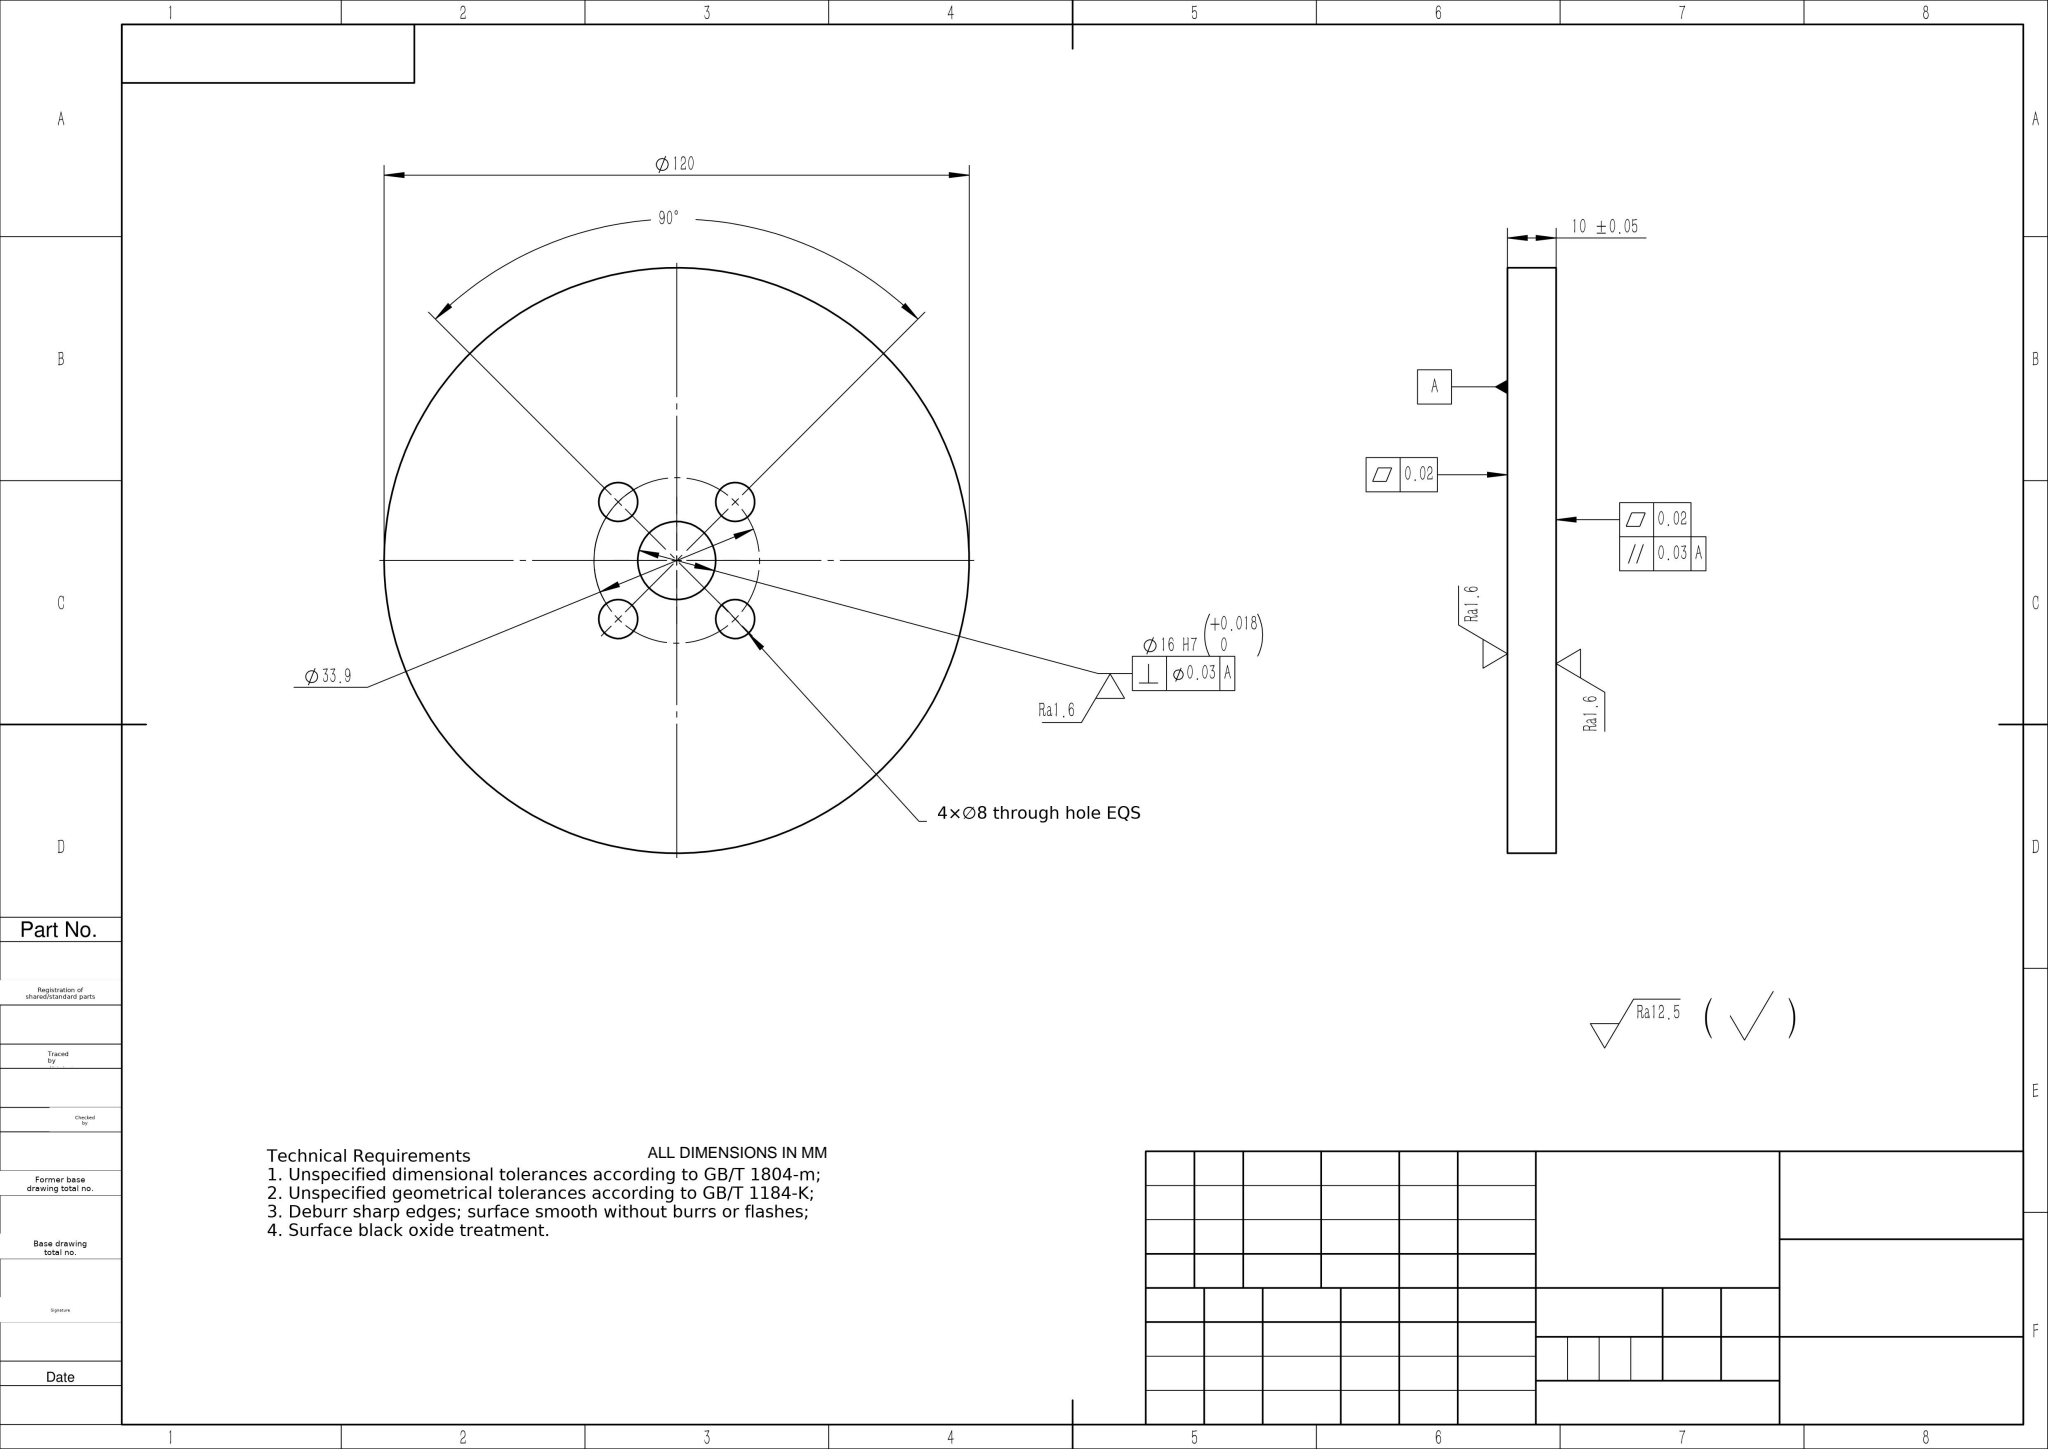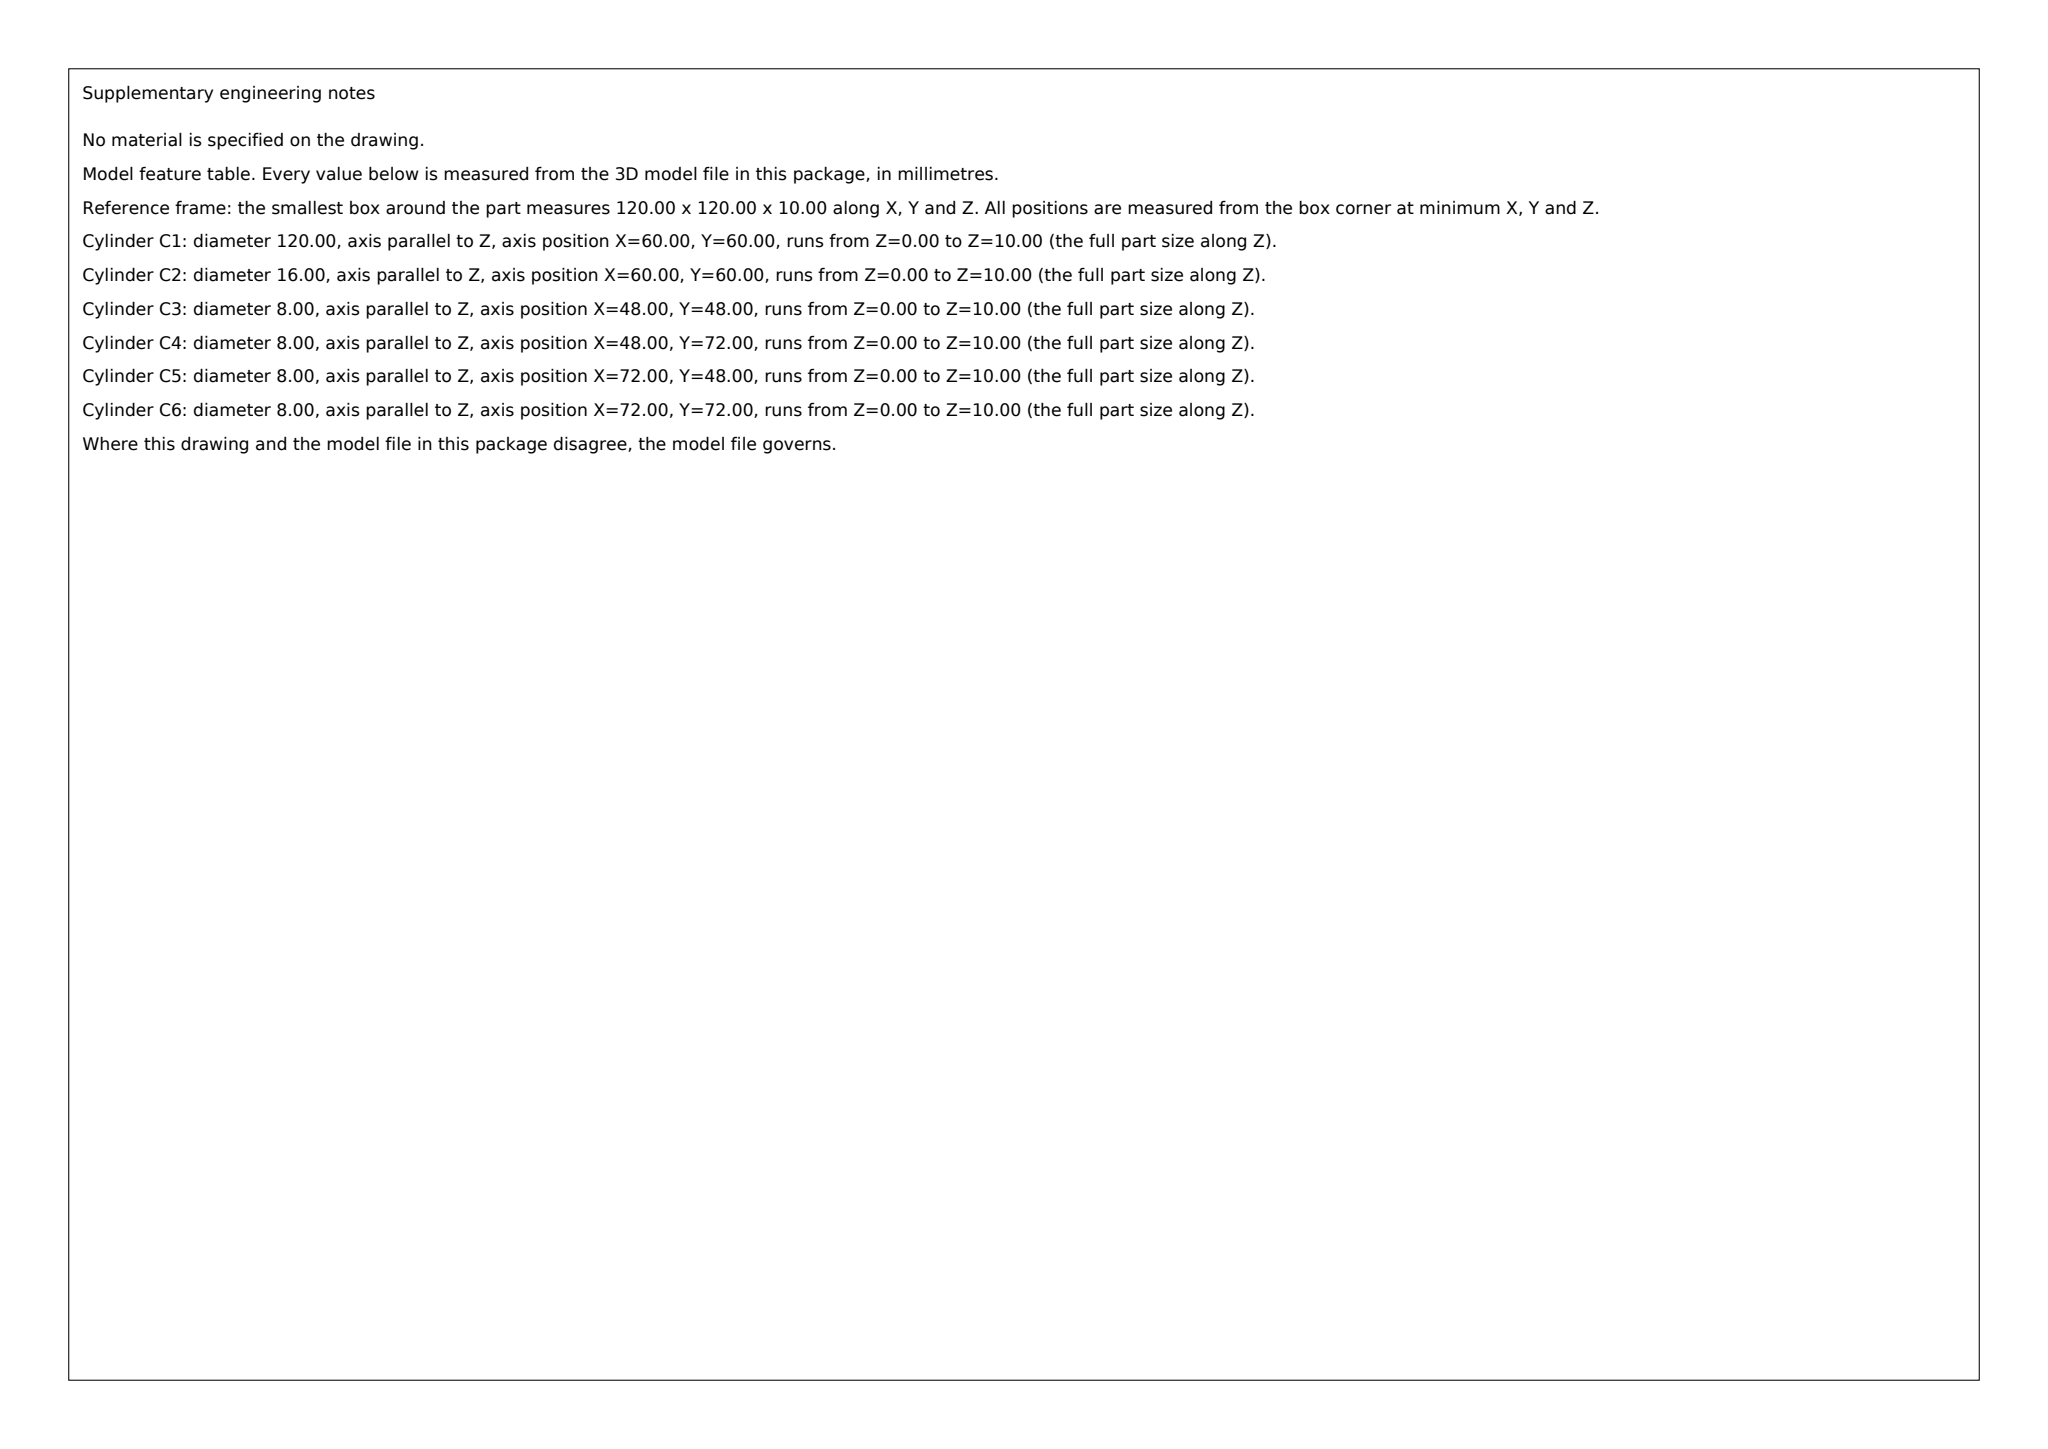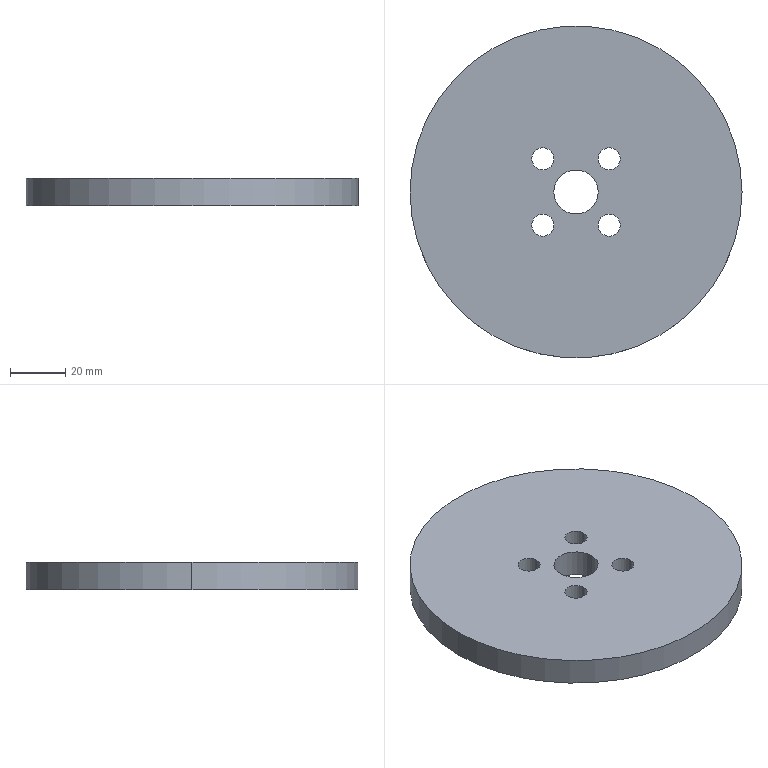Part | SolidWorks | mm | 1 solid | 14 faces | box 120 x 120 x 10 mm | volume 109076 mm3 | cylinder 12 | plane 2 | commonest cylinder face diameters 8 x8 16 x2 120 x2
build123d program:
from build123d import *

# Parameters (mm, degrees)
SKETCH1_R           = 20
BOSS_EXTRUDE1_DEPTH = 5
SKETCH2_R           = 30
BOSS_EXTRUDE2_DEPTH = 5
CUT_EXTRUDE1_REACH  = 44.72
SKETCH3_R           = 2
CUT_EXTRUDE3_REACH  = 44.72
SKETCH5_R           = 4
SCALE1_SCALE        = 2


with BuildPart() as part:
    # Sketch1 → Boss-Extrude1 (new body)
    with BuildSketch(Plane.XY):
        Circle(SKETCH1_R)
    extrude(amount=BOSS_EXTRUDE1_DEPTH)

    # Sketch2 → Boss-Extrude2 (add)
    with BuildSketch(Plane.XY.offset(5)):
        Circle(SKETCH2_R)
    extrude(amount=-BOSS_EXTRUDE2_DEPTH)

    # Sketch3 → Cut-Extrude1 (cut, up to next)
    with BuildSketch(Plane.XY.offset(5), mode=Mode.PRIVATE) as cut_extrude1_sk1:
        with Locations((-6, 6)):
            Circle(SKETCH3_R)
    cut_extrude1_tool1 = extrude(cut_extrude1_sk1.sketch, amount=-CUT_EXTRUDE1_REACH, mode=Mode.PRIVATE) & part.part
    # Sketch3 → Cut-Extrude1 (cut, up to next)
    with BuildSketch(Plane.XY.offset(5), mode=Mode.PRIVATE) as cut_extrude1_sk2:
        with Locations((-6, -6)):
            Circle(SKETCH3_R)
    cut_extrude1_tool2 = extrude(cut_extrude1_sk2.sketch, amount=-CUT_EXTRUDE1_REACH, mode=Mode.PRIVATE) & part.part
    # Sketch3 → Cut-Extrude1 (cut, up to next)
    with BuildSketch(Plane.XY.offset(5), mode=Mode.PRIVATE) as cut_extrude1_sk3:
        with Locations((6, -6)):
            Circle(SKETCH3_R)
    cut_extrude1_tool3 = extrude(cut_extrude1_sk3.sketch, amount=-CUT_EXTRUDE1_REACH, mode=Mode.PRIVATE) & part.part
    # Sketch3 → Cut-Extrude1 (cut, up to next)
    with BuildSketch(Plane.XY.offset(5), mode=Mode.PRIVATE) as cut_extrude1_sk4:
        with Locations((6, 6)):
            Circle(SKETCH3_R)
    cut_extrude1_tool4 = extrude(cut_extrude1_sk4.sketch, amount=-CUT_EXTRUDE1_REACH, mode=Mode.PRIVATE) & part.part
    add(cut_extrude1_tool1.solids().sort_by_distance((-6, 6, 5))[0], mode=Mode.SUBTRACT)
    add(cut_extrude1_tool2.solids().sort_by_distance((-6, -6, 5))[0], mode=Mode.SUBTRACT)
    add(cut_extrude1_tool3.solids().sort_by_distance((6, -6, 5))[0], mode=Mode.SUBTRACT)
    add(cut_extrude1_tool4.solids().sort_by_distance((6, 6, 5))[0], mode=Mode.SUBTRACT)

    # Sketch5 → Cut-Extrude3 (cut, up to next)
    with BuildSketch(Plane(origin=(0, 0, 0), x_dir=(-1, 0, 0), z_dir=(0, 0, -1)), mode=Mode.PRIVATE) as cut_extrude3_sk1:
        Circle(SKETCH5_R)
    cut_extrude3_tool1 = extrude(cut_extrude3_sk1.sketch, amount=-CUT_EXTRUDE3_REACH, mode=Mode.PRIVATE) & part.part
    add(cut_extrude3_tool1.solids().sort_by_distance((0, 0, 0))[0], mode=Mode.SUBTRACT)


with BuildPart() as part_1:
    # Scale1: scaled about (0, 0, 2.5)
    add(part.part.scale(SCALE1_SCALE).moved(Location((0, 0, -2.5))))


solid = part_1.part
STEP:
#1=CARTESIAN_POINT('',(8.,0.,7.5));
#2=VERTEX_POINT('',#1);
#3=CARTESIAN_POINT('',(-8.,0.,7.5));
#4=VERTEX_POINT('',#3);
#5=CARTESIAN_POINT('',(0.,0.,7.5));
#6=DIRECTION('',(0.,-0.,-1.));
#7=DIRECTION('',(1.,-0.,0.));
#8=AXIS2_PLACEMENT_3D('',#5,#6,#7);
#9=CIRCLE('',#8,8.);
#10=EDGE_CURVE('',#2,#4,#9,.T.);
#11=ORIENTED_EDGE('',*,*,#10,.F.);
#12=CARTESIAN_POINT('',(8.,0.,-2.5));
#13=VERTEX_POINT('',#12);
#14=CARTESIAN_POINT('',(8.,0.,7.502));
#15=DIRECTION('',(0.,-0.,-1.));
#16=VECTOR('',#15,1000.);
#17=LINE('',#14,#16);
#18=EDGE_CURVE('',#2,#13,#17,.T.);
#19=ORIENTED_EDGE('',*,*,#18,.T.);
#20=CARTESIAN_POINT('',(-8.,0.,-2.5));
#21=VERTEX_POINT('',#20);
#22=CARTESIAN_POINT('',(0.,0.,-2.5));
#23=DIRECTION('',(0.,-0.,-1.));
#24=DIRECTION('',(-1.,0.,0.));
#25=AXIS2_PLACEMENT_3D('',#22,#23,#24);
#26=CIRCLE('',#25,8.);
#27=EDGE_CURVE('',#13,#21,#26,.T.);
#28=ORIENTED_EDGE('',*,*,#27,.T.);
#29=CARTESIAN_POINT('',(-8.,0.,7.502));
#30=DIRECTION('',(0.,-0.,-1.));
#31=VECTOR('',#30,1000.);
#32=LINE('',#29,#31);
#33=EDGE_CURVE('',#4,#21,#32,.T.);
#34=ORIENTED_EDGE('',*,*,#33,.F.);
#35=EDGE_LOOP('',(#11,#19,#28,#34));
#36=FACE_OUTER_BOUND('',#35,.T.);
#37=CARTESIAN_POINT('',(0.,0.,7.502));
#38=DIRECTION('',(0.,-0.,-1.));
#39=DIRECTION('',(-1.,0.,0.));
#40=AXIS2_PLACEMENT_3D('',#37,#38,#39);
#41=CYLINDRICAL_SURFACE('',#40,8.);
#42=ADVANCED_FACE('',(#36),#41,.F.);
#43=CARTESIAN_POINT('',(16.,12.,-2.5));
#44=VERTEX_POINT('',#43);
#45=CARTESIAN_POINT('',(8.,12.,-2.5));
#46=VERTEX_POINT('',#45);
#47=CARTESIAN_POINT('',(12.,12.,-2.5));
#48=DIRECTION('',(0.,-0.,-1.));
#49=DIRECTION('',(1.,0.,0.));
#50=AXIS2_PLACEMENT_3D('',#47,#48,#49);
#51=CIRCLE('',#50,4.);
#52=EDGE_CURVE('',#44,#46,#51,.T.);
#53=ORIENTED_EDGE('',*,*,#52,.T.);
#54=CARTESIAN_POINT('',(8.,12.,7.5));
#55=VERTEX_POINT('',#54);
#56=CARTESIAN_POINT('',(8.,12.,-2.502));
#57=DIRECTION('',(-0.,0.,1.));
#58=VECTOR('',#57,1000.);
#59=LINE('',#56,#58);
#60=EDGE_CURVE('',#46,#55,#59,.T.);
#61=ORIENTED_EDGE('',*,*,#60,.T.);
#62=CARTESIAN_POINT('',(16.,12.,7.5));
#63=VERTEX_POINT('',#62);
#64=CARTESIAN_POINT('',(12.,12.,7.5));
#65=DIRECTION('',(-0.,0.,1.));
#66=DIRECTION('',(1.,0.,0.));
#67=AXIS2_PLACEMENT_3D('',#64,#65,#66);
#68=CIRCLE('',#67,4.);
#69=EDGE_CURVE('',#55,#63,#68,.T.);
#70=ORIENTED_EDGE('',*,*,#69,.T.);
#71=CARTESIAN_POINT('',(16.,12.,-2.502));
#72=DIRECTION('',(-0.,0.,1.));
#73=VECTOR('',#72,1000.);
#74=LINE('',#71,#73);
#75=EDGE_CURVE('',#44,#63,#74,.T.);
#76=ORIENTED_EDGE('',*,*,#75,.F.);
#77=EDGE_LOOP('',(#53,#61,#70,#76));
#78=FACE_OUTER_BOUND('',#77,.T.);
#79=CARTESIAN_POINT('',(12.,12.,-2.502));
#80=DIRECTION('',(-0.,0.,1.));
#81=DIRECTION('',(1.,0.,0.));
#82=AXIS2_PLACEMENT_3D('',#79,#80,#81);
#83=CYLINDRICAL_SURFACE('',#82,4.);
#84=ADVANCED_FACE('',(#78),#83,.F.);
#85=CARTESIAN_POINT('',(16.,-12.,-2.5));
#86=VERTEX_POINT('',#85);
#87=CARTESIAN_POINT('',(8.,-12.,-2.5));
#88=VERTEX_POINT('',#87);
#89=CARTESIAN_POINT('',(12.,-12.,-2.5));
#90=DIRECTION('',(0.,-0.,-1.));
#91=DIRECTION('',(1.,0.,0.));
#92=AXIS2_PLACEMENT_3D('',#89,#90,#91);
#93=CIRCLE('',#92,4.);
#94=EDGE_CURVE('',#86,#88,#93,.T.);
#95=ORIENTED_EDGE('',*,*,#94,.T.);
#96=CARTESIAN_POINT('',(8.,-12.,7.5));
#97=VERTEX_POINT('',#96);
#98=CARTESIAN_POINT('',(8.,-12.,-2.502));
#99=DIRECTION('',(-0.,0.,1.));
#100=VECTOR('',#99,1000.);
#101=LINE('',#98,#100);
#102=EDGE_CURVE('',#88,#97,#101,.T.);
#103=ORIENTED_EDGE('',*,*,#102,.T.);
#104=CARTESIAN_POINT('',(16.,-12.,7.5));
#105=VERTEX_POINT('',#104);
#106=CARTESIAN_POINT('',(12.,-12.,7.5));
#107=DIRECTION('',(-0.,0.,1.));
#108=DIRECTION('',(1.,0.,0.));
#109=AXIS2_PLACEMENT_3D('',#106,#107,#108);
#110=CIRCLE('',#109,4.);
#111=EDGE_CURVE('',#97,#105,#110,.T.);
#112=ORIENTED_EDGE('',*,*,#111,.T.);
#113=CARTESIAN_POINT('',(16.,-12.,-2.502));
#114=DIRECTION('',(-0.,0.,1.));
#115=VECTOR('',#114,1000.);
#116=LINE('',#113,#115);
#117=EDGE_CURVE('',#86,#105,#116,.T.);
#118=ORIENTED_EDGE('',*,*,#117,.F.);
#119=EDGE_LOOP('',(#95,#103,#112,#118));
#120=FACE_OUTER_BOUND('',#119,.T.);
#121=CARTESIAN_POINT('',(12.,-12.,-2.502));
#122=DIRECTION('',(-0.,0.,1.));
#123=DIRECTION('',(1.,0.,0.));
#124=AXIS2_PLACEMENT_3D('',#121,#122,#123);
#125=CYLINDRICAL_SURFACE('',#124,4.);
#126=ADVANCED_FACE('',(#120),#125,.F.);
#127=CARTESIAN_POINT('',(-8.,-12.,-2.5));
#128=VERTEX_POINT('',#127);
#129=CARTESIAN_POINT('',(-16.,-12.,-2.5));
#130=VERTEX_POINT('',#129);
#131=CARTESIAN_POINT('',(-12.,-12.,-2.5));
#132=DIRECTION('',(0.,-0.,-1.));
#133=DIRECTION('',(1.,0.,0.));
#134=AXIS2_PLACEMENT_3D('',#131,#132,#133);
#135=CIRCLE('',#134,4.);
#136=EDGE_CURVE('',#128,#130,#135,.T.);
#137=ORIENTED_EDGE('',*,*,#136,.T.);
#138=CARTESIAN_POINT('',(-16.,-12.,7.5));
#139=VERTEX_POINT('',#138);
#140=CARTESIAN_POINT('',(-16.,-12.,-2.502));
#141=DIRECTION('',(-0.,0.,1.));
#142=VECTOR('',#141,1000.);
#143=LINE('',#140,#142);
#144=EDGE_CURVE('',#130,#139,#143,.T.);
#145=ORIENTED_EDGE('',*,*,#144,.T.);
#146=CARTESIAN_POINT('',(-8.,-12.,7.5));
#147=VERTEX_POINT('',#146);
#148=CARTESIAN_POINT('',(-12.,-12.,7.5));
#149=DIRECTION('',(-0.,0.,1.));
#150=DIRECTION('',(1.,0.,0.));
#151=AXIS2_PLACEMENT_3D('',#148,#149,#150);
#152=CIRCLE('',#151,4.);
#153=EDGE_CURVE('',#139,#147,#152,.T.);
#154=ORIENTED_EDGE('',*,*,#153,.T.);
#155=CARTESIAN_POINT('',(-8.,-12.,-2.502));
#156=DIRECTION('',(-0.,0.,1.));
#157=VECTOR('',#156,1000.);
#158=LINE('',#155,#157);
#159=EDGE_CURVE('',#128,#147,#158,.T.);
#160=ORIENTED_EDGE('',*,*,#159,.F.);
#161=EDGE_LOOP('',(#137,#145,#154,#160));
#162=FACE_OUTER_BOUND('',#161,.T.);
#163=CARTESIAN_POINT('',(-12.,-12.,-2.502));
#164=DIRECTION('',(-0.,0.,1.));
#165=DIRECTION('',(1.,0.,0.));
#166=AXIS2_PLACEMENT_3D('',#163,#164,#165);
#167=CYLINDRICAL_SURFACE('',#166,4.);
#168=ADVANCED_FACE('',(#162),#167,.F.);
#169=CARTESIAN_POINT('',(-8.,12.,-2.5));
#170=VERTEX_POINT('',#169);
#171=CARTESIAN_POINT('',(-16.,12.,-2.5));
#172=VERTEX_POINT('',#171);
#173=CARTESIAN_POINT('',(-12.,12.,-2.5));
#174=DIRECTION('',(0.,-0.,-1.));
#175=DIRECTION('',(1.,0.,0.));
#176=AXIS2_PLACEMENT_3D('',#173,#174,#175);
#177=CIRCLE('',#176,4.);
#178=EDGE_CURVE('',#170,#172,#177,.T.);
#179=ORIENTED_EDGE('',*,*,#178,.T.);
#180=CARTESIAN_POINT('',(-16.,12.,7.5));
#181=VERTEX_POINT('',#180);
#182=CARTESIAN_POINT('',(-16.,12.,-2.502));
#183=DIRECTION('',(-0.,0.,1.));
#184=VECTOR('',#183,1000.);
#185=LINE('',#182,#184);
#186=EDGE_CURVE('',#172,#181,#185,.T.);
#187=ORIENTED_EDGE('',*,*,#186,.T.);
#188=CARTESIAN_POINT('',(-8.,12.,7.5));
#189=VERTEX_POINT('',#188);
#190=CARTESIAN_POINT('',(-12.,12.,7.5));
#191=DIRECTION('',(-0.,0.,1.));
#192=DIRECTION('',(1.,0.,0.));
#193=AXIS2_PLACEMENT_3D('',#190,#191,#192);
#194=CIRCLE('',#193,4.);
#195=EDGE_CURVE('',#181,#189,#194,.T.);
#196=ORIENTED_EDGE('',*,*,#195,.T.);
#197=CARTESIAN_POINT('',(-8.,12.,-2.502));
#198=DIRECTION('',(-0.,0.,1.));
#199=VECTOR('',#198,1000.);
#200=LINE('',#197,#199);
#201=EDGE_CURVE('',#170,#189,#200,.T.);
#202=ORIENTED_EDGE('',*,*,#201,.F.);
#203=EDGE_LOOP('',(#179,#187,#196,#202));
#204=FACE_OUTER_BOUND('',#203,.T.);
#205=CARTESIAN_POINT('',(-12.,12.,-2.502));
#206=DIRECTION('',(-0.,0.,1.));
#207=DIRECTION('',(1.,0.,0.));
#208=AXIS2_PLACEMENT_3D('',#205,#206,#207);
#209=CYLINDRICAL_SURFACE('',#208,4.);
#210=ADVANCED_FACE('',(#204),#209,.F.);
#211=CARTESIAN_POINT('',(60.,-0.,-2.5));
#212=VERTEX_POINT('',#211);
#213=CARTESIAN_POINT('',(-60.,0.,-2.5));
#214=VERTEX_POINT('',#213);
#215=CARTESIAN_POINT('',(0.,0.,-2.5));
#216=DIRECTION('',(-0.,0.,1.));
#217=DIRECTION('',(1.,-0.,0.));
#218=AXIS2_PLACEMENT_3D('',#215,#216,#217);
#219=CIRCLE('',#218,60.);
#220=EDGE_CURVE('',#212,#214,#219,.T.);
#221=ORIENTED_EDGE('',*,*,#220,.T.);
#222=CARTESIAN_POINT('',(-60.,0.,7.5));
#223=VERTEX_POINT('',#222);
#224=CARTESIAN_POINT('',(-60.,0.,-2.5));
#225=DIRECTION('',(-0.,0.,1.));
#226=VECTOR('',#225,1000.);
#227=LINE('',#224,#226);
#228=EDGE_CURVE('',#214,#223,#227,.T.);
#229=ORIENTED_EDGE('',*,*,#228,.T.);
#230=CARTESIAN_POINT('',(60.,-0.,7.5));
#231=VERTEX_POINT('',#230);
#232=CARTESIAN_POINT('',(0.,0.,7.5));
#233=DIRECTION('',(-0.,0.,1.));
#234=DIRECTION('',(1.,-0.,0.));
#235=AXIS2_PLACEMENT_3D('',#232,#233,#234);
#236=CIRCLE('',#235,60.);
#237=EDGE_CURVE('',#231,#223,#236,.T.);
#238=ORIENTED_EDGE('',*,*,#237,.F.);
#239=CARTESIAN_POINT('',(60.,-0.,-2.5));
#240=DIRECTION('',(-0.,0.,1.));
#241=VECTOR('',#240,1000.);
#242=LINE('',#239,#241);
#243=EDGE_CURVE('',#212,#231,#242,.T.);
#244=ORIENTED_EDGE('',*,*,#243,.F.);
#245=EDGE_LOOP('',(#221,#229,#238,#244));
#246=FACE_OUTER_BOUND('',#245,.T.);
#247=CARTESIAN_POINT('',(0.,0.,-2.5));
#248=DIRECTION('',(-0.,0.,1.));
#249=DIRECTION('',(1.,-0.,0.));
#250=AXIS2_PLACEMENT_3D('',#247,#248,#249);
#251=CYLINDRICAL_SURFACE('',#250,60.);
#252=ADVANCED_FACE('',(#246),#251,.T.);
#253=CARTESIAN_POINT('',(0.,0.,-2.5));
#254=DIRECTION('',(0.,-0.,-1.));
#255=DIRECTION('',(-1.,0.,0.));
#256=AXIS2_PLACEMENT_3D('',#253,#254,#255);
#257=CIRCLE('',#256,8.);
#258=EDGE_CURVE('',#21,#13,#257,.T.);
#259=ORIENTED_EDGE('',*,*,#258,.F.);
#260=ORIENTED_EDGE('',*,*,#27,.F.);
#261=EDGE_LOOP('',(#259,#260));
#262=FACE_BOUND('',#261,.T.);
#263=ORIENTED_EDGE('',*,*,#52,.F.);
#264=CARTESIAN_POINT('',(12.,12.,-2.5));
#265=DIRECTION('',(0.,-0.,-1.));
#266=DIRECTION('',(1.,0.,0.));
#267=AXIS2_PLACEMENT_3D('',#264,#265,#266);
#268=CIRCLE('',#267,4.);
#269=EDGE_CURVE('',#46,#44,#268,.T.);
#270=ORIENTED_EDGE('',*,*,#269,.F.);
#271=EDGE_LOOP('',(#263,#270));
#272=FACE_BOUND('',#271,.T.);
#273=ORIENTED_EDGE('',*,*,#94,.F.);
#274=CARTESIAN_POINT('',(12.,-12.,-2.5));
#275=DIRECTION('',(0.,-0.,-1.));
#276=DIRECTION('',(1.,0.,0.));
#277=AXIS2_PLACEMENT_3D('',#274,#275,#276);
#278=CIRCLE('',#277,4.);
#279=EDGE_CURVE('',#88,#86,#278,.T.);
#280=ORIENTED_EDGE('',*,*,#279,.F.);
#281=EDGE_LOOP('',(#273,#280));
#282=FACE_BOUND('',#281,.T.);
#283=ORIENTED_EDGE('',*,*,#136,.F.);
#284=CARTESIAN_POINT('',(-12.,-12.,-2.5));
#285=DIRECTION('',(0.,-0.,-1.));
#286=DIRECTION('',(1.,0.,0.));
#287=AXIS2_PLACEMENT_3D('',#284,#285,#286);
#288=CIRCLE('',#287,4.);
#289=EDGE_CURVE('',#130,#128,#288,.T.);
#290=ORIENTED_EDGE('',*,*,#289,.F.);
#291=EDGE_LOOP('',(#283,#290));
#292=FACE_BOUND('',#291,.T.);
#293=ORIENTED_EDGE('',*,*,#178,.F.);
#294=CARTESIAN_POINT('',(-12.,12.,-2.5));
#295=DIRECTION('',(0.,-0.,-1.));
#296=DIRECTION('',(1.,0.,0.));
#297=AXIS2_PLACEMENT_3D('',#294,#295,#296);
#298=CIRCLE('',#297,4.);
#299=EDGE_CURVE('',#172,#170,#298,.T.);
#300=ORIENTED_EDGE('',*,*,#299,.F.);
#301=EDGE_LOOP('',(#293,#300));
#302=FACE_BOUND('',#301,.T.);
#303=ORIENTED_EDGE('',*,*,#220,.F.);
#304=CARTESIAN_POINT('',(0.,0.,-2.5));
#305=DIRECTION('',(-0.,0.,1.));
#306=DIRECTION('',(1.,-0.,0.));
#307=AXIS2_PLACEMENT_3D('',#304,#305,#306);
#308=CIRCLE('',#307,60.);
#309=EDGE_CURVE('',#214,#212,#308,.T.);
#310=ORIENTED_EDGE('',*,*,#309,.F.);
#311=EDGE_LOOP('',(#303,#310));
#312=FACE_OUTER_BOUND('',#311,.T.);
#313=CARTESIAN_POINT('',(0.,0.,-2.5));
#314=DIRECTION('',(0.,0.,1.));
#315=DIRECTION('',(1.,-0.,-0.));
#316=AXIS2_PLACEMENT_3D('',#313,#314,#315);
#317=PLANE('',#316);
#318=ADVANCED_FACE('',(#262,#272,#282,#292,#302,#312),#317,.F.);
#319=ORIENTED_EDGE('',*,*,#228,.F.);
#320=ORIENTED_EDGE('',*,*,#309,.T.);
#321=ORIENTED_EDGE('',*,*,#243,.T.);
#322=CARTESIAN_POINT('',(0.,0.,7.5));
#323=DIRECTION('',(-0.,0.,1.));
#324=DIRECTION('',(1.,-0.,0.));
#325=AXIS2_PLACEMENT_3D('',#322,#323,#324);
#326=CIRCLE('',#325,60.);
#327=EDGE_CURVE('',#223,#231,#326,.T.);
#328=ORIENTED_EDGE('',*,*,#327,.F.);
#329=EDGE_LOOP('',(#319,#320,#321,#328));
#330=FACE_OUTER_BOUND('',#329,.T.);
#331=CARTESIAN_POINT('',(0.,0.,-2.5));
#332=DIRECTION('',(-0.,0.,1.));
#333=DIRECTION('',(1.,-0.,0.));
#334=AXIS2_PLACEMENT_3D('',#331,#332,#333);
#335=CYLINDRICAL_SURFACE('',#334,60.);
#336=ADVANCED_FACE('',(#330),#335,.T.);
#337=CARTESIAN_POINT('',(0.,0.,7.5));
#338=DIRECTION('',(0.,-0.,-1.));
#339=DIRECTION('',(1.,-0.,0.));
#340=AXIS2_PLACEMENT_3D('',#337,#338,#339);
#341=CIRCLE('',#340,8.);
#342=EDGE_CURVE('',#4,#2,#341,.T.);
#343=ORIENTED_EDGE('',*,*,#342,.T.);
#344=ORIENTED_EDGE('',*,*,#10,.T.);
#345=EDGE_LOOP('',(#343,#344));
#346=FACE_BOUND('',#345,.T.);
#347=CARTESIAN_POINT('',(12.,12.,7.5));
#348=DIRECTION('',(-0.,0.,1.));
#349=DIRECTION('',(1.,0.,0.));
#350=AXIS2_PLACEMENT_3D('',#347,#348,#349);
#351=CIRCLE('',#350,4.);
#352=EDGE_CURVE('',#63,#55,#351,.T.);
#353=ORIENTED_EDGE('',*,*,#352,.F.);
#354=ORIENTED_EDGE('',*,*,#69,.F.);
#355=EDGE_LOOP('',(#353,#354));
#356=FACE_BOUND('',#355,.T.);
#357=CARTESIAN_POINT('',(12.,-12.,7.5));
#358=DIRECTION('',(-0.,0.,1.));
#359=DIRECTION('',(1.,0.,0.));
#360=AXIS2_PLACEMENT_3D('',#357,#358,#359);
#361=CIRCLE('',#360,4.);
#362=EDGE_CURVE('',#105,#97,#361,.T.);
#363=ORIENTED_EDGE('',*,*,#362,.F.);
#364=ORIENTED_EDGE('',*,*,#111,.F.);
#365=EDGE_LOOP('',(#363,#364));
#366=FACE_BOUND('',#365,.T.);
#367=CARTESIAN_POINT('',(-12.,-12.,7.5));
#368=DIRECTION('',(-0.,0.,1.));
#369=DIRECTION('',(1.,0.,0.));
#370=AXIS2_PLACEMENT_3D('',#367,#368,#369);
#371=CIRCLE('',#370,4.);
#372=EDGE_CURVE('',#147,#139,#371,.T.);
#373=ORIENTED_EDGE('',*,*,#372,.F.);
#374=ORIENTED_EDGE('',*,*,#153,.F.);
#375=EDGE_LOOP('',(#373,#374));
#376=FACE_BOUND('',#375,.T.);
#377=CARTESIAN_POINT('',(-12.,12.,7.5));
#378=DIRECTION('',(-0.,0.,1.));
#379=DIRECTION('',(1.,0.,0.));
#380=AXIS2_PLACEMENT_3D('',#377,#378,#379);
#381=CIRCLE('',#380,4.);
#382=EDGE_CURVE('',#189,#181,#381,.T.);
#383=ORIENTED_EDGE('',*,*,#382,.F.);
#384=ORIENTED_EDGE('',*,*,#195,.F.);
#385=EDGE_LOOP('',(#383,#384));
#386=FACE_BOUND('',#385,.T.);
#387=ORIENTED_EDGE('',*,*,#237,.T.);
#388=ORIENTED_EDGE('',*,*,#327,.T.);
#389=EDGE_LOOP('',(#387,#388));
#390=FACE_OUTER_BOUND('',#389,.T.);
#391=CARTESIAN_POINT('',(0.,0.,7.5));
#392=DIRECTION('',(0.,0.,1.));
#393=DIRECTION('',(1.,-0.,-0.));
#394=AXIS2_PLACEMENT_3D('',#391,#392,#393);
#395=PLANE('',#394);
#396=ADVANCED_FACE('',(#346,#356,#366,#376,#386,#390),#395,.T.);
#397=ORIENTED_EDGE('',*,*,#186,.F.);
#398=ORIENTED_EDGE('',*,*,#299,.T.);
#399=ORIENTED_EDGE('',*,*,#201,.T.);
#400=ORIENTED_EDGE('',*,*,#382,.T.);
#401=EDGE_LOOP('',(#397,#398,#399,#400));
#402=FACE_OUTER_BOUND('',#401,.T.);
#403=CARTESIAN_POINT('',(-12.,12.,-2.502));
#404=DIRECTION('',(-0.,0.,1.));
#405=DIRECTION('',(1.,0.,0.));
#406=AXIS2_PLACEMENT_3D('',#403,#404,#405);
#407=CYLINDRICAL_SURFACE('',#406,4.);
#408=ADVANCED_FACE('',(#402),#407,.F.);
#409=ORIENTED_EDGE('',*,*,#144,.F.);
#410=ORIENTED_EDGE('',*,*,#289,.T.);
#411=ORIENTED_EDGE('',*,*,#159,.T.);
#412=ORIENTED_EDGE('',*,*,#372,.T.);
#413=EDGE_LOOP('',(#409,#410,#411,#412));
#414=FACE_OUTER_BOUND('',#413,.T.);
#415=CARTESIAN_POINT('',(-12.,-12.,-2.502));
#416=DIRECTION('',(-0.,0.,1.));
#417=DIRECTION('',(1.,0.,0.));
#418=AXIS2_PLACEMENT_3D('',#415,#416,#417);
#419=CYLINDRICAL_SURFACE('',#418,4.);
#420=ADVANCED_FACE('',(#414),#419,.F.);
#421=ORIENTED_EDGE('',*,*,#102,.F.);
#422=ORIENTED_EDGE('',*,*,#279,.T.);
#423=ORIENTED_EDGE('',*,*,#117,.T.);
#424=ORIENTED_EDGE('',*,*,#362,.T.);
#425=EDGE_LOOP('',(#421,#422,#423,#424));
#426=FACE_OUTER_BOUND('',#425,.T.);
#427=CARTESIAN_POINT('',(12.,-12.,-2.502));
#428=DIRECTION('',(-0.,0.,1.));
#429=DIRECTION('',(1.,0.,0.));
#430=AXIS2_PLACEMENT_3D('',#427,#428,#429);
#431=CYLINDRICAL_SURFACE('',#430,4.);
#432=ADVANCED_FACE('',(#426),#431,.F.);
#433=ORIENTED_EDGE('',*,*,#60,.F.);
#434=ORIENTED_EDGE('',*,*,#269,.T.);
#435=ORIENTED_EDGE('',*,*,#75,.T.);
#436=ORIENTED_EDGE('',*,*,#352,.T.);
#437=EDGE_LOOP('',(#433,#434,#435,#436));
#438=FACE_OUTER_BOUND('',#437,.T.);
#439=CARTESIAN_POINT('',(12.,12.,-2.502));
#440=DIRECTION('',(-0.,0.,1.));
#441=DIRECTION('',(1.,0.,0.));
#442=AXIS2_PLACEMENT_3D('',#439,#440,#441);
#443=CYLINDRICAL_SURFACE('',#442,4.);
#444=ADVANCED_FACE('',(#438),#443,.F.);
#445=ORIENTED_EDGE('',*,*,#18,.F.);
#446=ORIENTED_EDGE('',*,*,#342,.F.);
#447=ORIENTED_EDGE('',*,*,#33,.T.);
#448=ORIENTED_EDGE('',*,*,#258,.T.);
#449=EDGE_LOOP('',(#445,#446,#447,#448));
#450=FACE_OUTER_BOUND('',#449,.T.);
#451=CARTESIAN_POINT('',(0.,0.,7.502));
#452=DIRECTION('',(0.,-0.,-1.));
#453=DIRECTION('',(-1.,0.,0.));
#454=AXIS2_PLACEMENT_3D('',#451,#452,#453);
#455=CYLINDRICAL_SURFACE('',#454,8.);
#456=ADVANCED_FACE('',(#450),#455,.F.);
#457=CLOSED_SHELL('',(#42,#84,#126,#168,#210,#252,#318,#336,#396,#408,#420,#432,#444,#456));
#458=MANIFOLD_SOLID_BREP('',#457);
#459=CARTESIAN_POINT('',(0.,0.,0.));
#460=DIRECTION('',(0.,0.,1.));
#461=DIRECTION('',(1.,0.,0.));
#462=AXIS2_PLACEMENT_3D('',#459,#460,#461);
#463=(LENGTH_UNIT()NAMED_UNIT(*)SI_UNIT(.MILLI.,.METRE.));
#464=UNCERTAINTY_MEASURE_WITH_UNIT(LENGTH_MEASURE(0.00001),#463,'','');
#465=(NAMED_UNIT(*)PLANE_ANGLE_UNIT()SI_UNIT($,.RADIAN.));
#466=(NAMED_UNIT(*)SI_UNIT($,.STERADIAN.)SOLID_ANGLE_UNIT());
#467=(GEOMETRIC_REPRESENTATION_CONTEXT(3)GLOBAL_UNCERTAINTY_ASSIGNED_CONTEXT((#464))GLOBAL_UNIT_ASSIGNED_CONTEXT((#463,#465,#466))REPRESENTATION_CONTEXT('',''));
#468=ADVANCED_BREP_SHAPE_REPRESENTATION('',(#458,#462),#467);